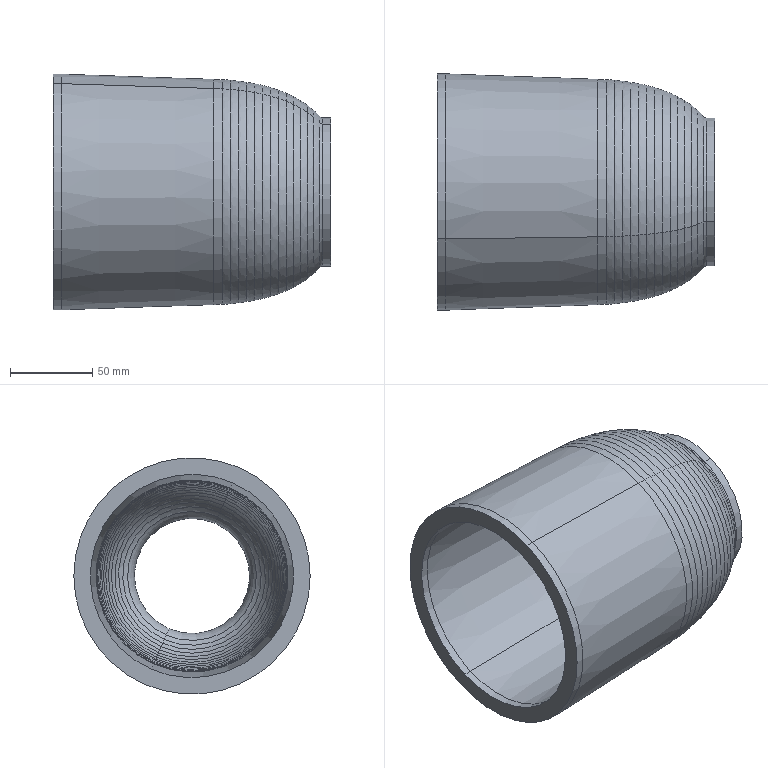Component | SolidWorks | EdgeTrimmingWorkpieceMold-1 | 1 solid | 74 faces | box 168.61 x 143.54 x 143.54 mm | volume 663861 mm3 | torus 56 | cone 8 | cylinder 8 | plane 2 | commonest cylinder face diameters 123.537 x2 143.537 x2 89.98 x2 69.98 x2
build123d program:
from build123d import *


with BuildPart() as part:
    # Model → Revolve1 (revolve)
    with BuildSketch(Plane.XY, mode=Mode.PRIVATE) as revolve1_sk:
        with BuildLine():
            Line((15157.55, -1332.763), (15157.55, -1327.763))
            Line((15157.55, -1327.763), (15147.55, -1327.763))
            Line((15147.55, -1327.763), (15147.55, -1332.763))
            ThreePointArc((15147.55, -1332.763), (15147.346, -1333.71), (15146.77, -1334.489))
            ThreePointArc((15146.77, -1334.489), (15144.903, -1336.225), (15143.13, -1338.058))
            ThreePointArc((15143.13, -1338.058), (15141.502, -1339.923), (15139.966, -1341.865))
            ThreePointArc((15139.966, -1341.865), (15138.514, -1343.885), (15137.152, -1345.967))
            ThreePointArc((15137.152, -1345.967), (15135.876, -1348.11), (15134.686, -1350.301))
            ThreePointArc((15134.686, -1350.301), (15133.577, -1352.538), (15132.547, -1354.814))
            ThreePointArc((15132.547, -1354.814), (15131.593, -1357.123), (15130.711, -1359.462))
            ThreePointArc((15130.711, -1359.462), (15129.898, -1361.827), (15129.151, -1364.213))
            ThreePointArc((15129.151, -1364.213), (15128.465, -1366.618), (15127.839, -1369.04))
            ThreePointArc((15127.839, -1369.04), (15127.269, -1371.476), (15126.753, -1373.924))
            ThreePointArc((15126.753, -1373.924), (15126.287, -1376.382), (15125.869, -1378.849))
            ThreePointArc((15125.869, -1378.849), (15125.497, -1381.323), (15125.169, -1383.804))
            ThreePointArc((15125.169, -1383.804), (15124.882, -1386.29), (15124.634, -1388.78))
            ThreePointArc((15124.634, -1388.78), (15124.424, -1391.273), (15124.251, -1393.77))
            Line((15124.251, -1393.77), (15123.997, -1399.001))
            Line((15123.997, -1399.001), (15120.771, -1491.37))
            Line((15120.771, -1491.37), (15120.771, -1496.37))
            Line((15120.771, -1496.37), (15130.771, -1496.37))
            Line((15130.771, -1496.37), (15130.771, -1491.544))
            Line((15130.771, -1491.544), (15133.989, -1399.417))
            Line((15133.989, -1399.417), (15134.236, -1394.324))
            ThreePointArc((15134.236, -1394.324), (15134.398, -1392.006), (15134.593, -1389.69))
            ThreePointArc((15134.593, -1389.69), (15134.824, -1387.358), (15135.093, -1385.03))
            ThreePointArc((15135.093, -1385.03), (15135.399, -1382.723), (15135.745, -1380.423))
            ThreePointArc((15135.745, -1380.423), (15136.13, -1378.148), (15136.559, -1375.882))
            ThreePointArc((15136.559, -1375.882), (15137.031, -1373.648), (15137.551, -1371.424))
            ThreePointArc((15137.551, -1371.424), (15138.116, -1369.24), (15138.734, -1367.07))
            ThreePointArc((15138.734, -1367.07), (15139.399, -1364.947), (15140.122, -1362.844))
            ThreePointArc((15140.122, -1362.844), (15140.894, -1360.797), (15141.729, -1358.776))
            ThreePointArc((15141.729, -1358.776), (15142.613, -1356.821), (15143.566, -1354.9))
            ThreePointArc((15143.566, -1354.9), (15144.567, -1353.056), (15145.641, -1351.254))
            ThreePointArc((15145.641, -1351.254), (15146.761, -1349.541), (15147.956, -1347.879))
            ThreePointArc((15147.956, -1347.879), (15149.192, -1346.315), (15150.503, -1344.814))
            ThreePointArc((15150.503, -1344.814), (15151.904, -1343.365), (15153.38, -1341.993))
            ThreePointArc((15153.38, -1341.993), (15156.459, -1337.827), (15157.55, -1332.763))
        make_face()
    revolve(revolve1_sk.sketch.rotate(Axis((15192.54, -1249.447, 0), (0, -1, 0)), 270), axis=Axis((15192.54, -1249.447, 0), (0, -1, 0)))


solid = part.part

# Placed as in the assembly
solid = solid.moved(Location((1497.627, 16492.246, 687.116), (0, 0, -90)))